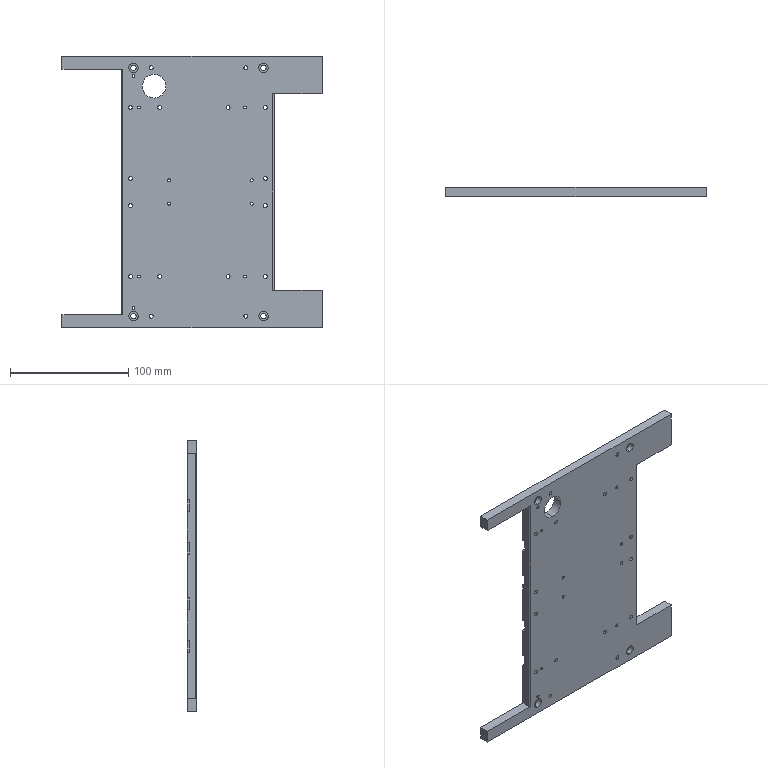CAM job | Mastercam | mm | 2 operations | part box 220 x 8 x 230
1. Contour (2D) | 12 - 12 平铣刀
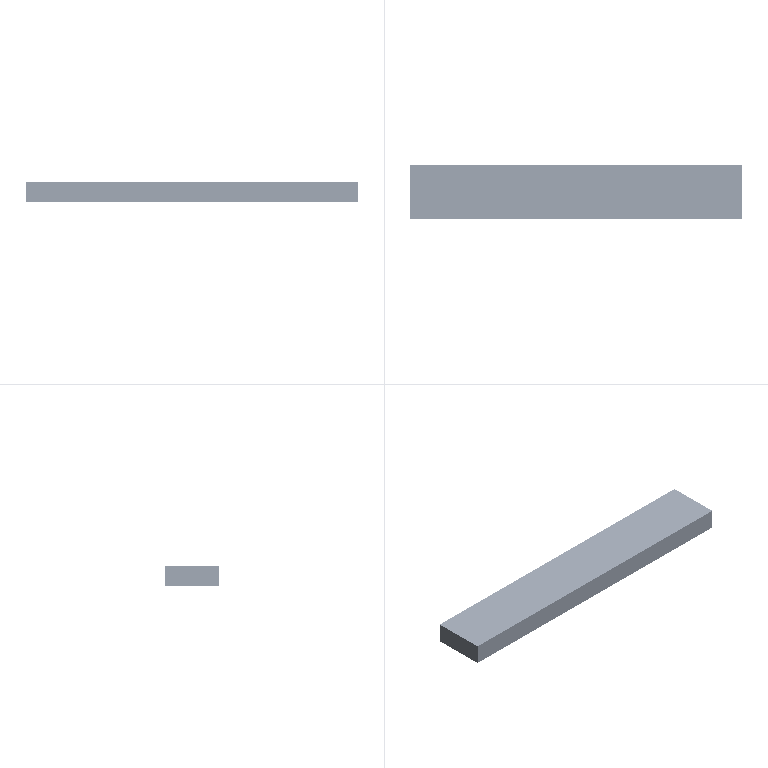2. Contour (2D) | 12 - 12 平铣刀